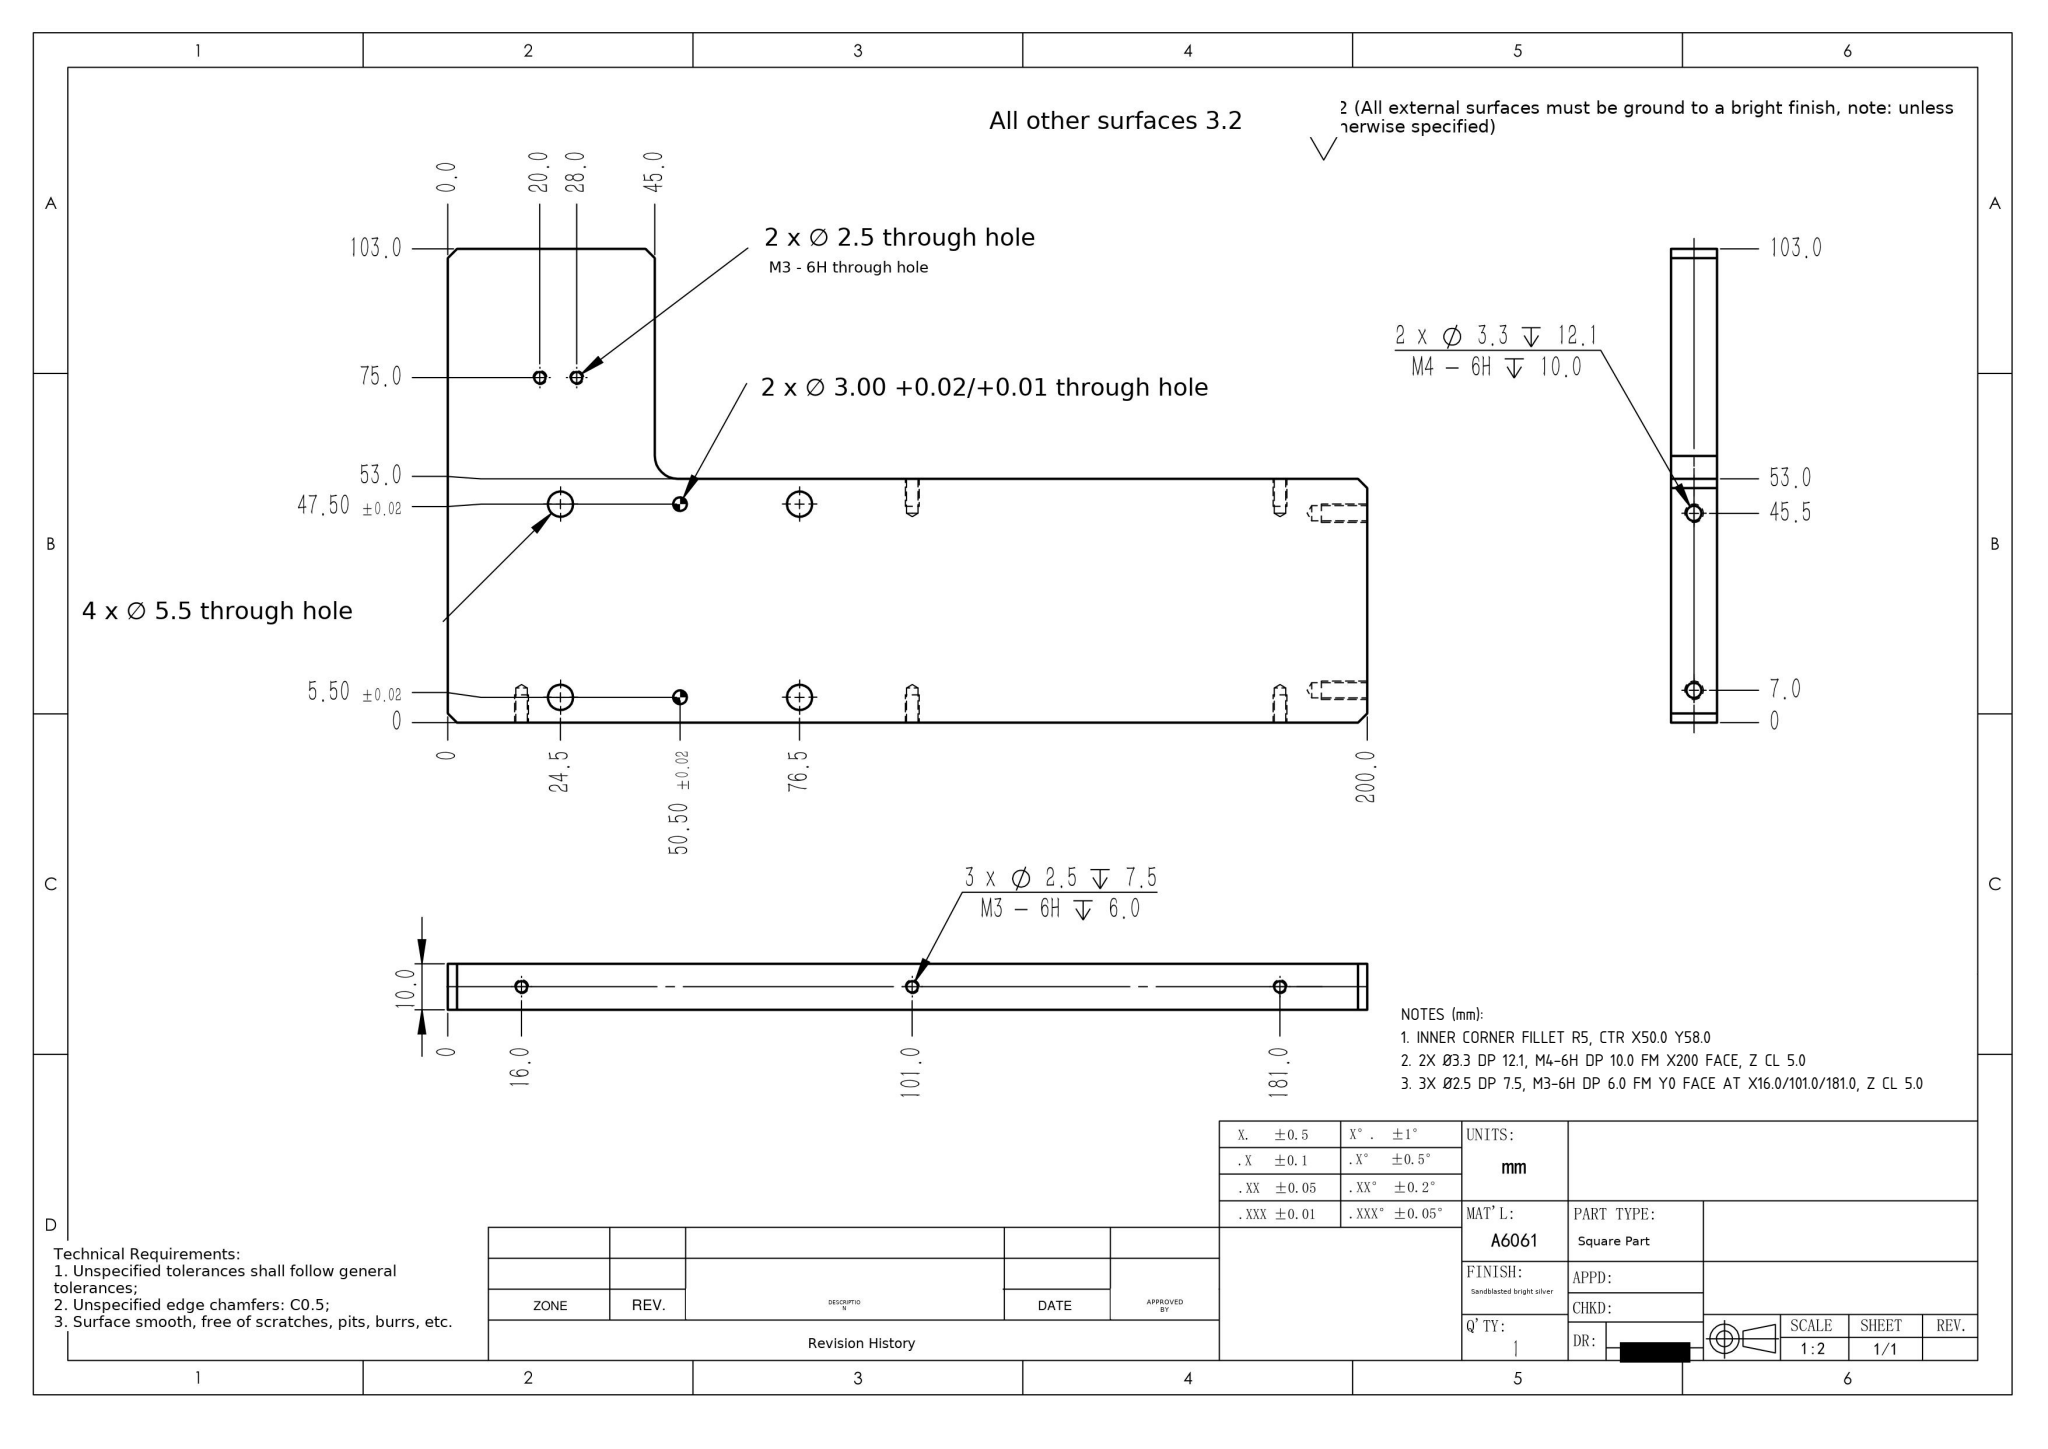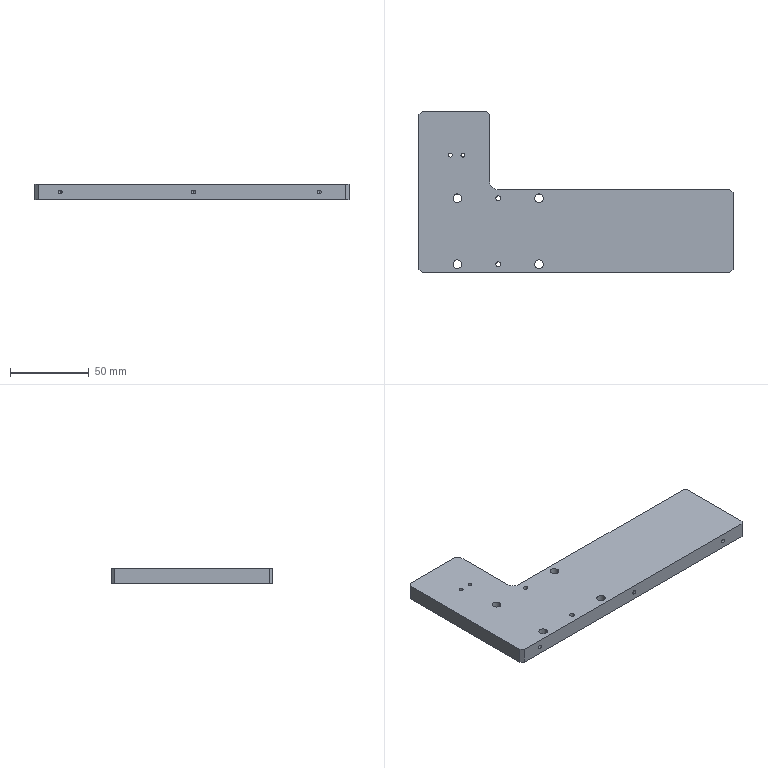Part | SolidWorks | mm | 1 solid | 58 faces | box 200 x 103 x 10 mm | volume 126861 mm3 | cylinder 31 | cone 14 | plane 13 | commonest cylinder face diameters 2.5 x14 5.5 x8 3.3 x4 3 x4 10 x1
Drawing notes:
INNER CORNER FILLET R5, CTR X50.0 Y58.0 | from the solid: cyl dia 10.0 axis z at (50.0,58.0), L=10 -> R5 tangent to planes x=45.0 & y=53.0
2X Ø3.3 DP 12.1, M4-6H DP 10.0 FM X200 FACE, Z CL 5.0 | from the solid: cyl dia 3.3 axis x len 12.1 at y=7.0 & 45.5, z=5.0, from plane x=200.0; cones 118 deg
3X Ø2.5 DP 7.5, M3-6H DP 6.0 FM Y0 FACE AT X16.0/101.0/181.0, Z CL 5.0 | from the solid: cyl dia 2.5 axis y len 7.5 at x=16.0,101.0,181.0, z=5.0, start plane y=0.0
build123d program:
from build123d import *

# Parameters (mm, degrees)
SKETCH1_W                  = 200
SKETCH1_H                  = 53
BOSS_EXTRUDE1_DEPTH        = 10
SKETCH2_W                  = 45
SKETCH2_H                  = 10
BOSS_EXTRUDE2_DEPTH        = 50
M3_TAPPED_HOLE1_D          = 2.5
M3_TAPPED_HOLE1_DEPTH      = 7.5
M3_TAPPED_HOLE1_TIP        = 0.7511
M3_TAPPED_HOLE2_D          = 2.5
M3_TAPPED_HOLE2_DEPTH      = 7.5
M3_TAPPED_HOLE2_TIP        = 0.7511
M5_CLEARANCE_HOLE_1_D      = 5.5
SIZE_MM_DOWEL_PIN_HOLE_1_D = 3
M3_TAPPED_HOLE3_D          = 2.5
M4_TAPPED_HOLE1_D          = 3.3
M4_TAPPED_HOLE1_DEPTH      = 12.1
M4_TAPPED_HOLE1_TIP        = 0.9914
FILLET1_R                  = 5
CHAMFER1_SIZE              = 2


with BuildPart() as part:
    # Sketch1 → Boss-Extrude1 (new body)
    with BuildSketch(Plane.XY):
        Rectangle(SKETCH1_W, SKETCH1_H)
    extrude(amount=BOSS_EXTRUDE1_DEPTH)

    # Sketch2 → Boss-Extrude2 (add)
    with BuildSketch(Plane(origin=(0, 26.5, 0), x_dir=(1, 0, 0), z_dir=(0, 1, 0))):
        with Locations((-77.5, -5)):
            Rectangle(SKETCH2_W, SKETCH2_H)
    extrude(amount=BOSS_EXTRUDE2_DEPTH)

    # M3 Tapped Hole1
    with Locations(Plane(origin=(0, -26.5, 0), x_dir=(-1, 0, 0), z_dir=(0, -1, 0))):
        with Locations((84, -5), (-1, -5), (-81, -5)):
            Hole(M3_TAPPED_HOLE1_D / 2, depth=M3_TAPPED_HOLE1_DEPTH)
            with Locations((0, 0, -(M3_TAPPED_HOLE1_DEPTH + M3_TAPPED_HOLE1_TIP / 2))):  # 118° drill point
                Cone(0, M3_TAPPED_HOLE1_D / 2, M3_TAPPED_HOLE1_TIP, mode=Mode.SUBTRACT)

    # M3 Tapped Hole2
    with Locations(Plane(origin=(0, 26.5, 0), x_dir=(1, 0, 0), z_dir=(0, 1, 0))):
        with Locations((1, -5), (81, -5)):
            Hole(M3_TAPPED_HOLE2_D / 2, depth=M3_TAPPED_HOLE2_DEPTH)
            with Locations((0, 0, -(M3_TAPPED_HOLE2_DEPTH + M3_TAPPED_HOLE2_TIP / 2))):  # 118° drill point
                Cone(0, M3_TAPPED_HOLE2_D / 2, M3_TAPPED_HOLE2_TIP, mode=Mode.SUBTRACT)

    # M5 Clearance Hole 1 (through all)
    with Locations(Plane.XY.offset(10)):
        with Locations((-75.5, -21), (-75.5, 21), (-23.5, 21), (-23.5, -21)):
            Hole(M5_CLEARANCE_HOLE_1_D / 2)

    # Size mm Dowel Pin Hole 1 (through all)
    with Locations(Plane.XY.offset(10)):
        with Locations((-49.5, 21), (-49.5, -21)):
            Hole(SIZE_MM_DOWEL_PIN_HOLE_1_D / 2)

    # M3 Tapped Hole3 (through all)
    with Locations(Plane.XY.offset(10)):
        with Locations((-72, 48.5), (-80, 48.5)):
            Hole(M3_TAPPED_HOLE3_D / 2)

    # M4 Tapped Hole1
    with Locations(Plane(origin=(100, 0, 0), x_dir=(0, 0, -1), z_dir=(1, 0, 0))):
        with Locations((-5, 19), (-5, -19.5)):
            Hole(M4_TAPPED_HOLE1_D / 2, depth=M4_TAPPED_HOLE1_DEPTH)
            with Locations((0, 0, -(M4_TAPPED_HOLE1_DEPTH + M4_TAPPED_HOLE1_TIP / 2))):  # 118° drill point
                Cone(0, M4_TAPPED_HOLE1_D / 2, M4_TAPPED_HOLE1_TIP, mode=Mode.SUBTRACT)

    # Fillet1
    fillet1_edges = [part.edges().sort_by_distance(p)[0] for p in [
        (-55, 26.5, 5),
    ]]
    fillet(fillet1_edges, radius=FILLET1_R)

    # Chamfer1
    chamfer1_edges = [part.edges().sort_by_distance(p)[0] for p in [
        (-100, 76.5, 5),
        (-55, 76.5, 5),
        (100, -26.5, 5),
        (-100, -26.5, 5),
        (100, 26.5, 5),
    ]]
    chamfer(chamfer1_edges, length=CHAMFER1_SIZE)


solid = part.part